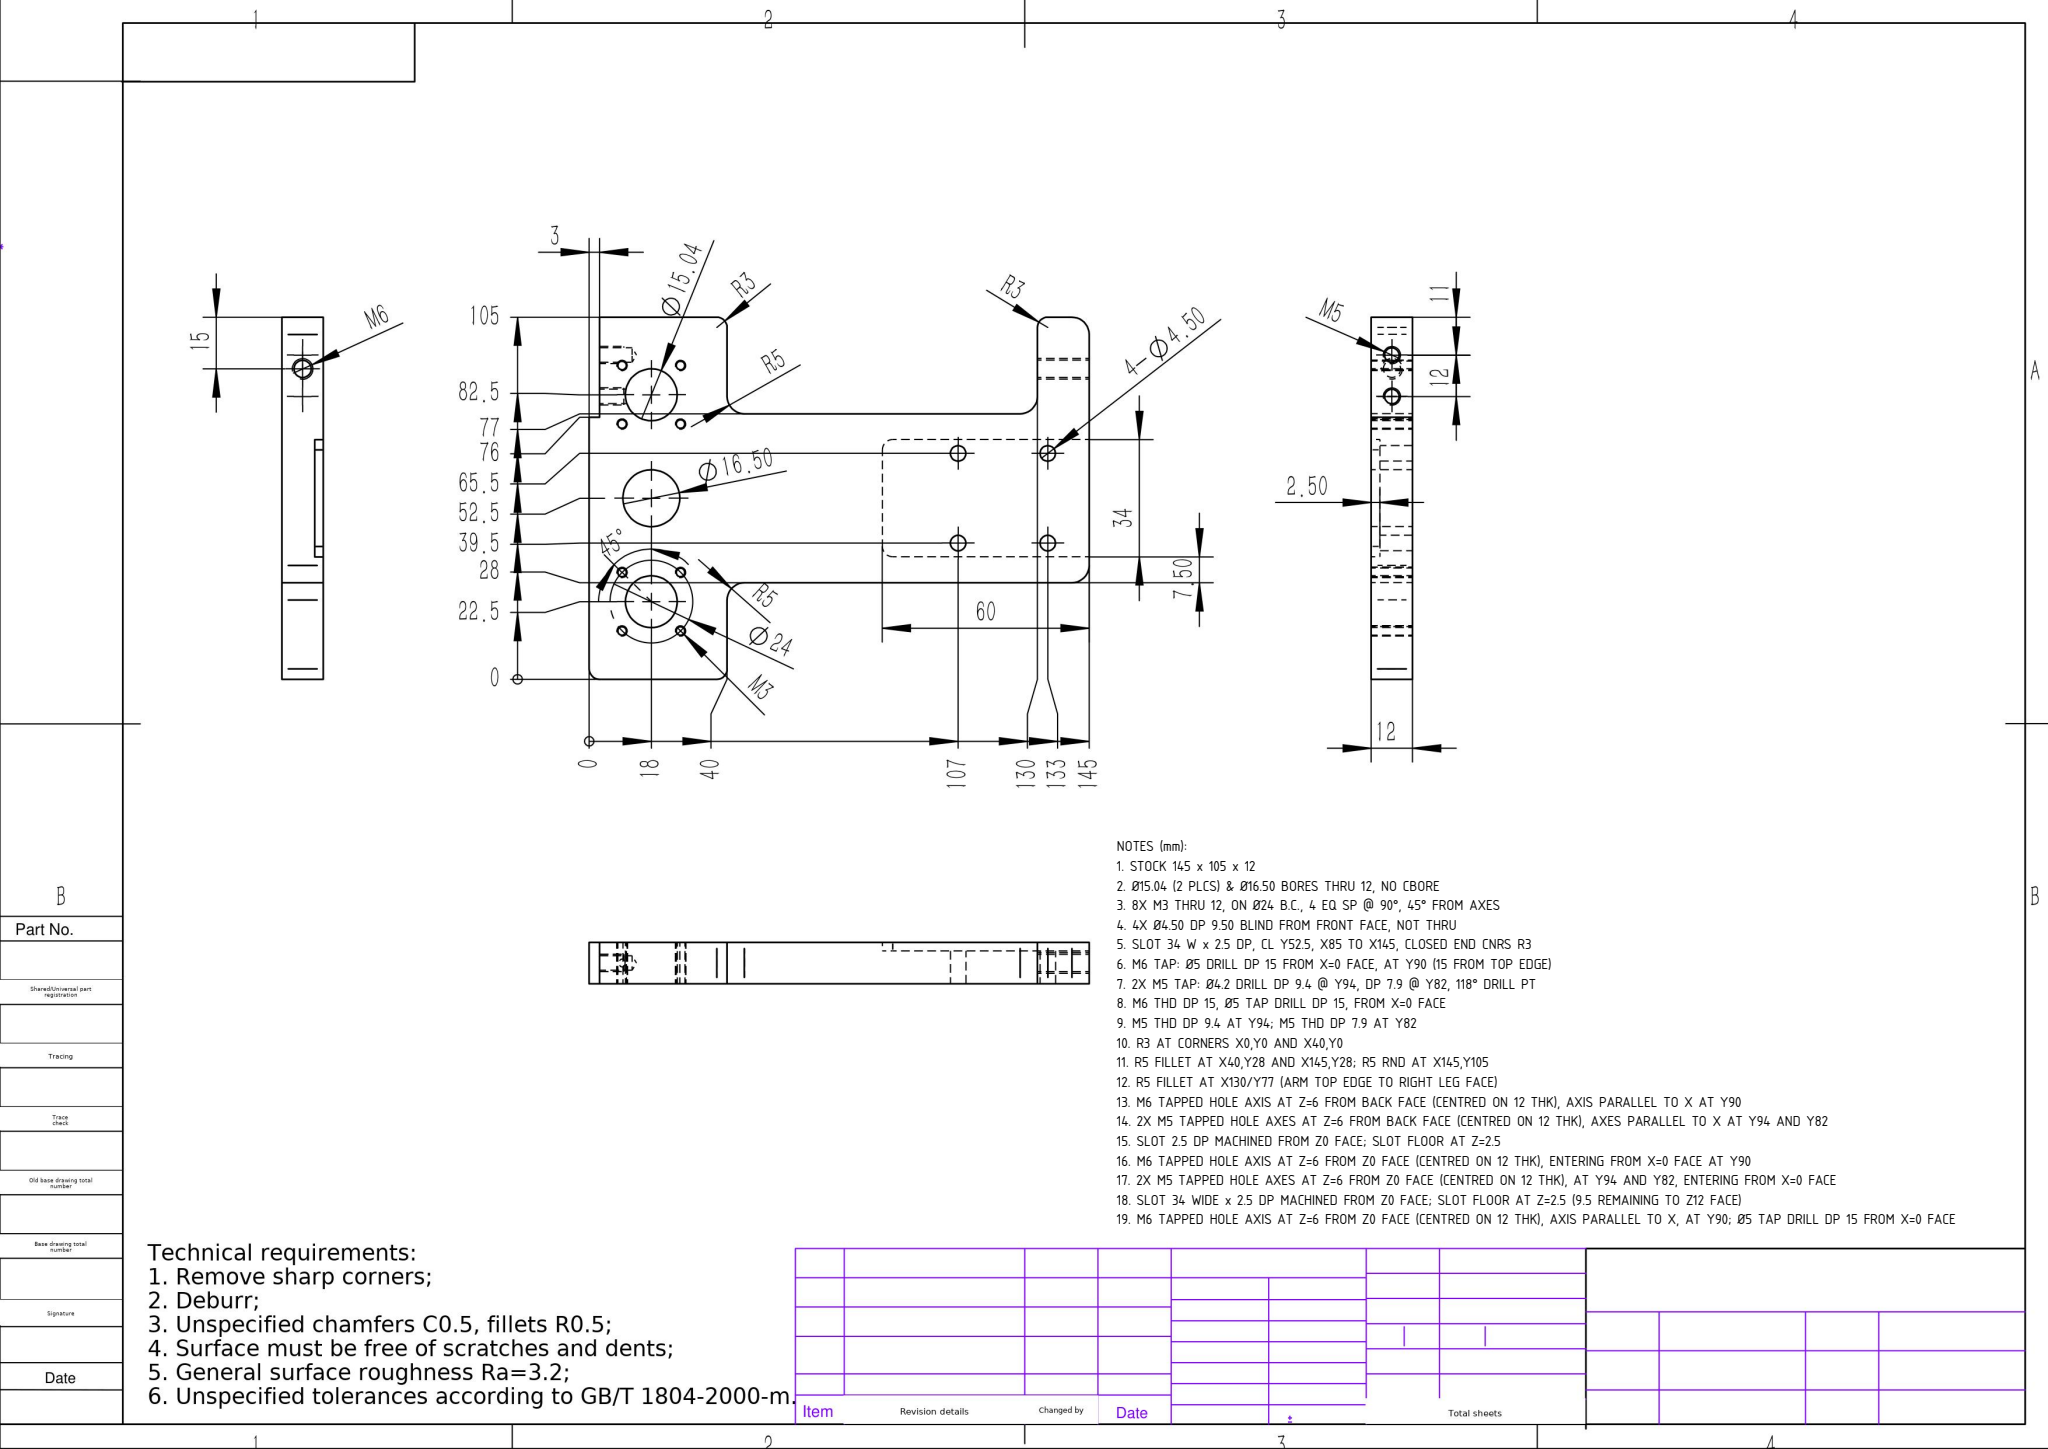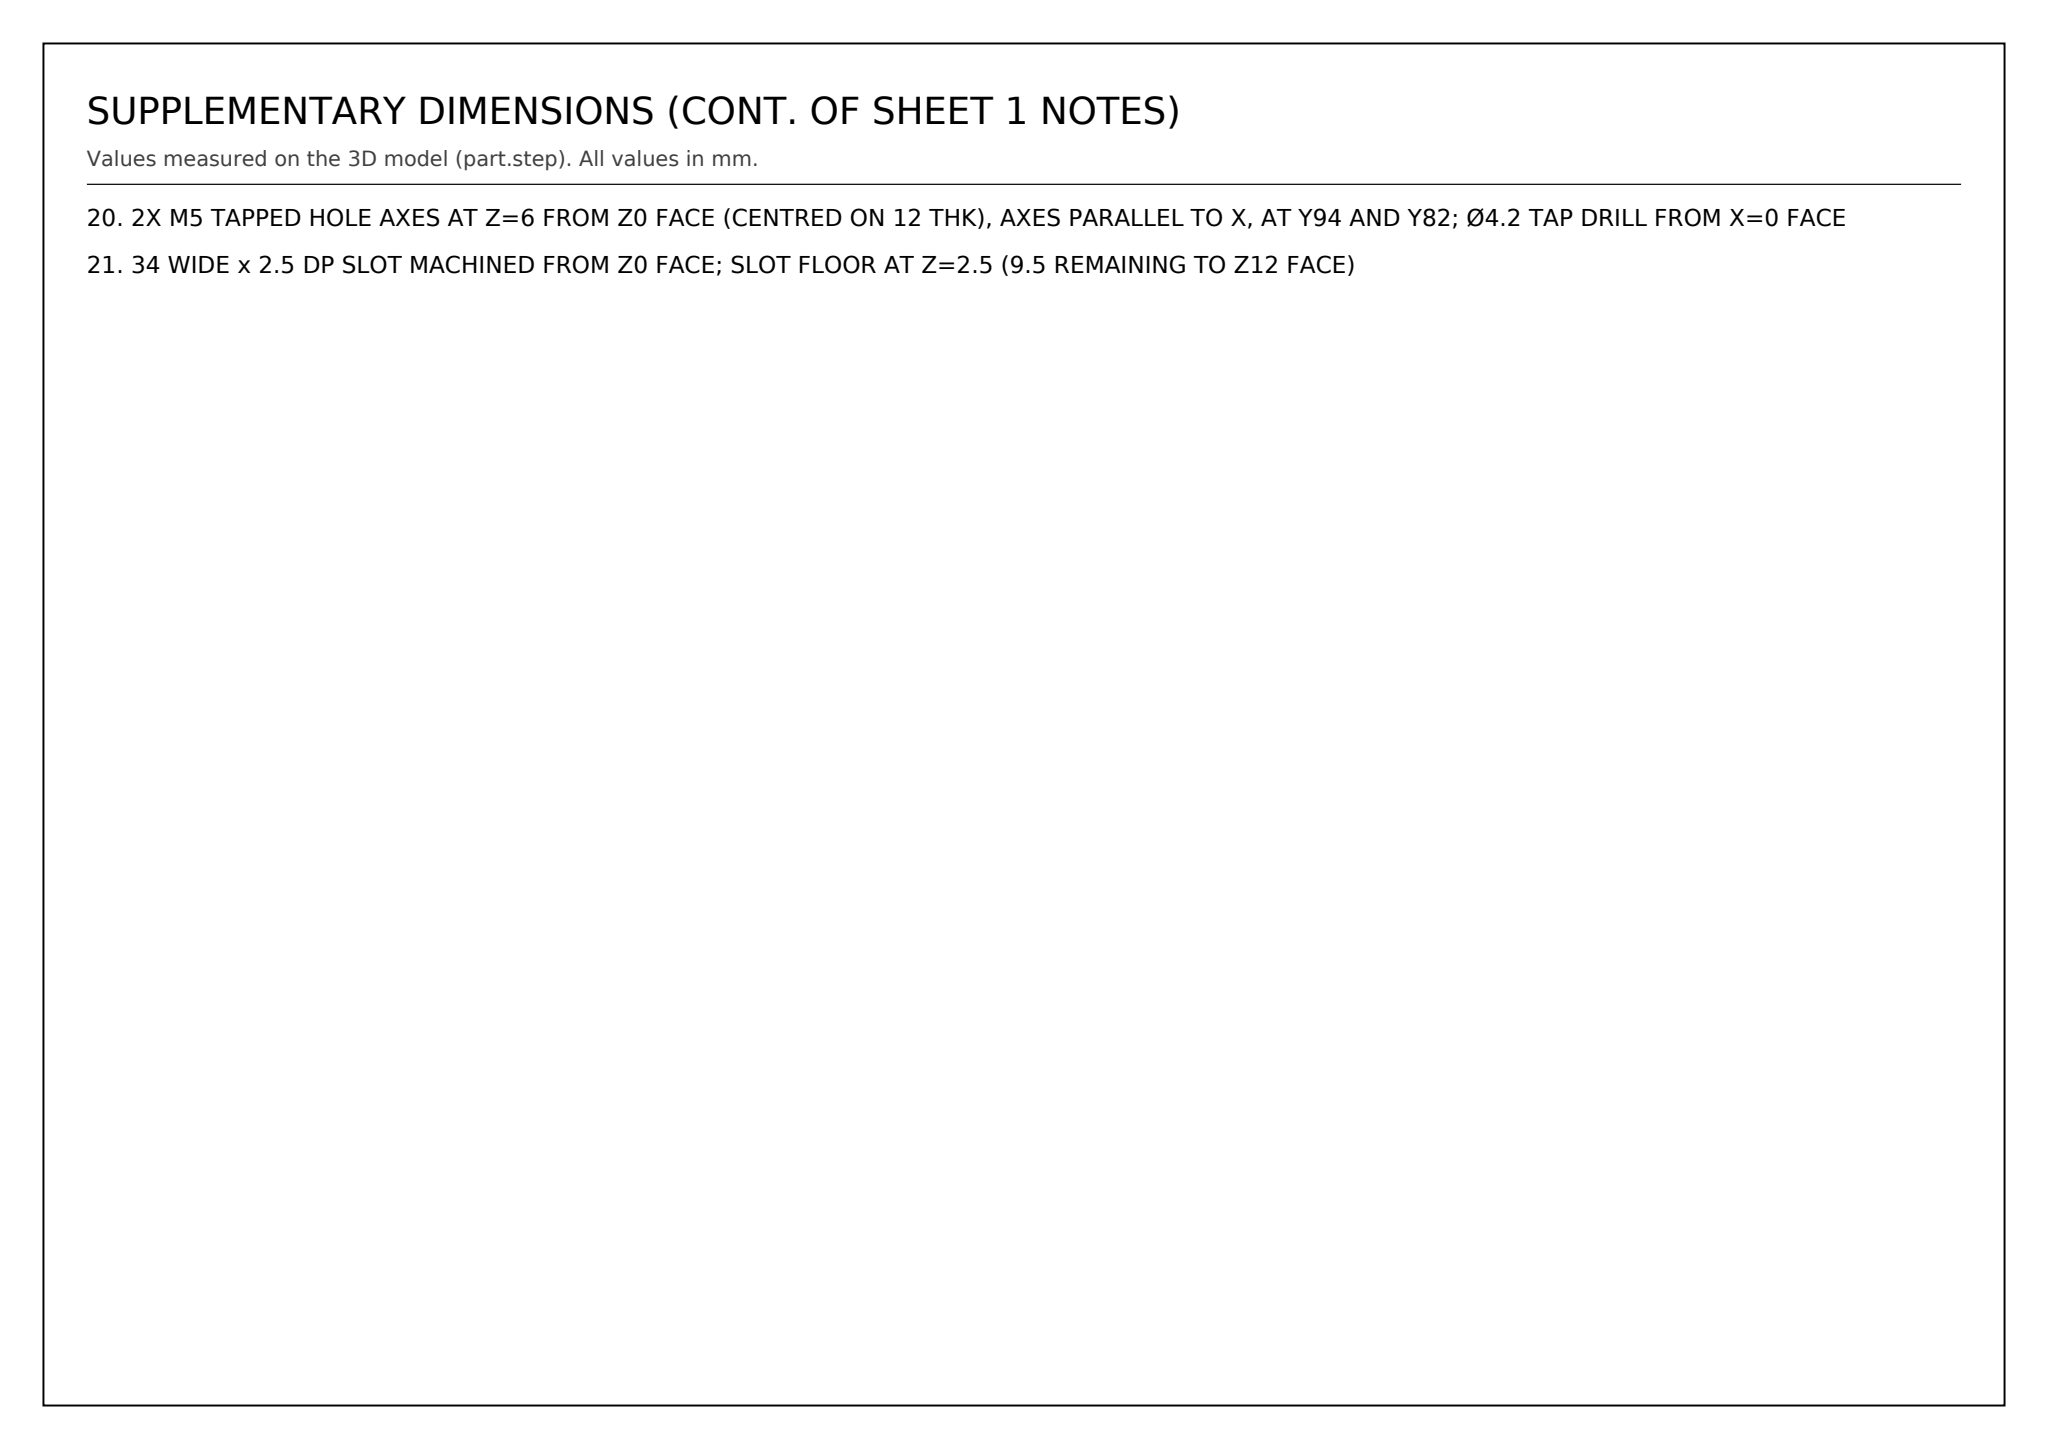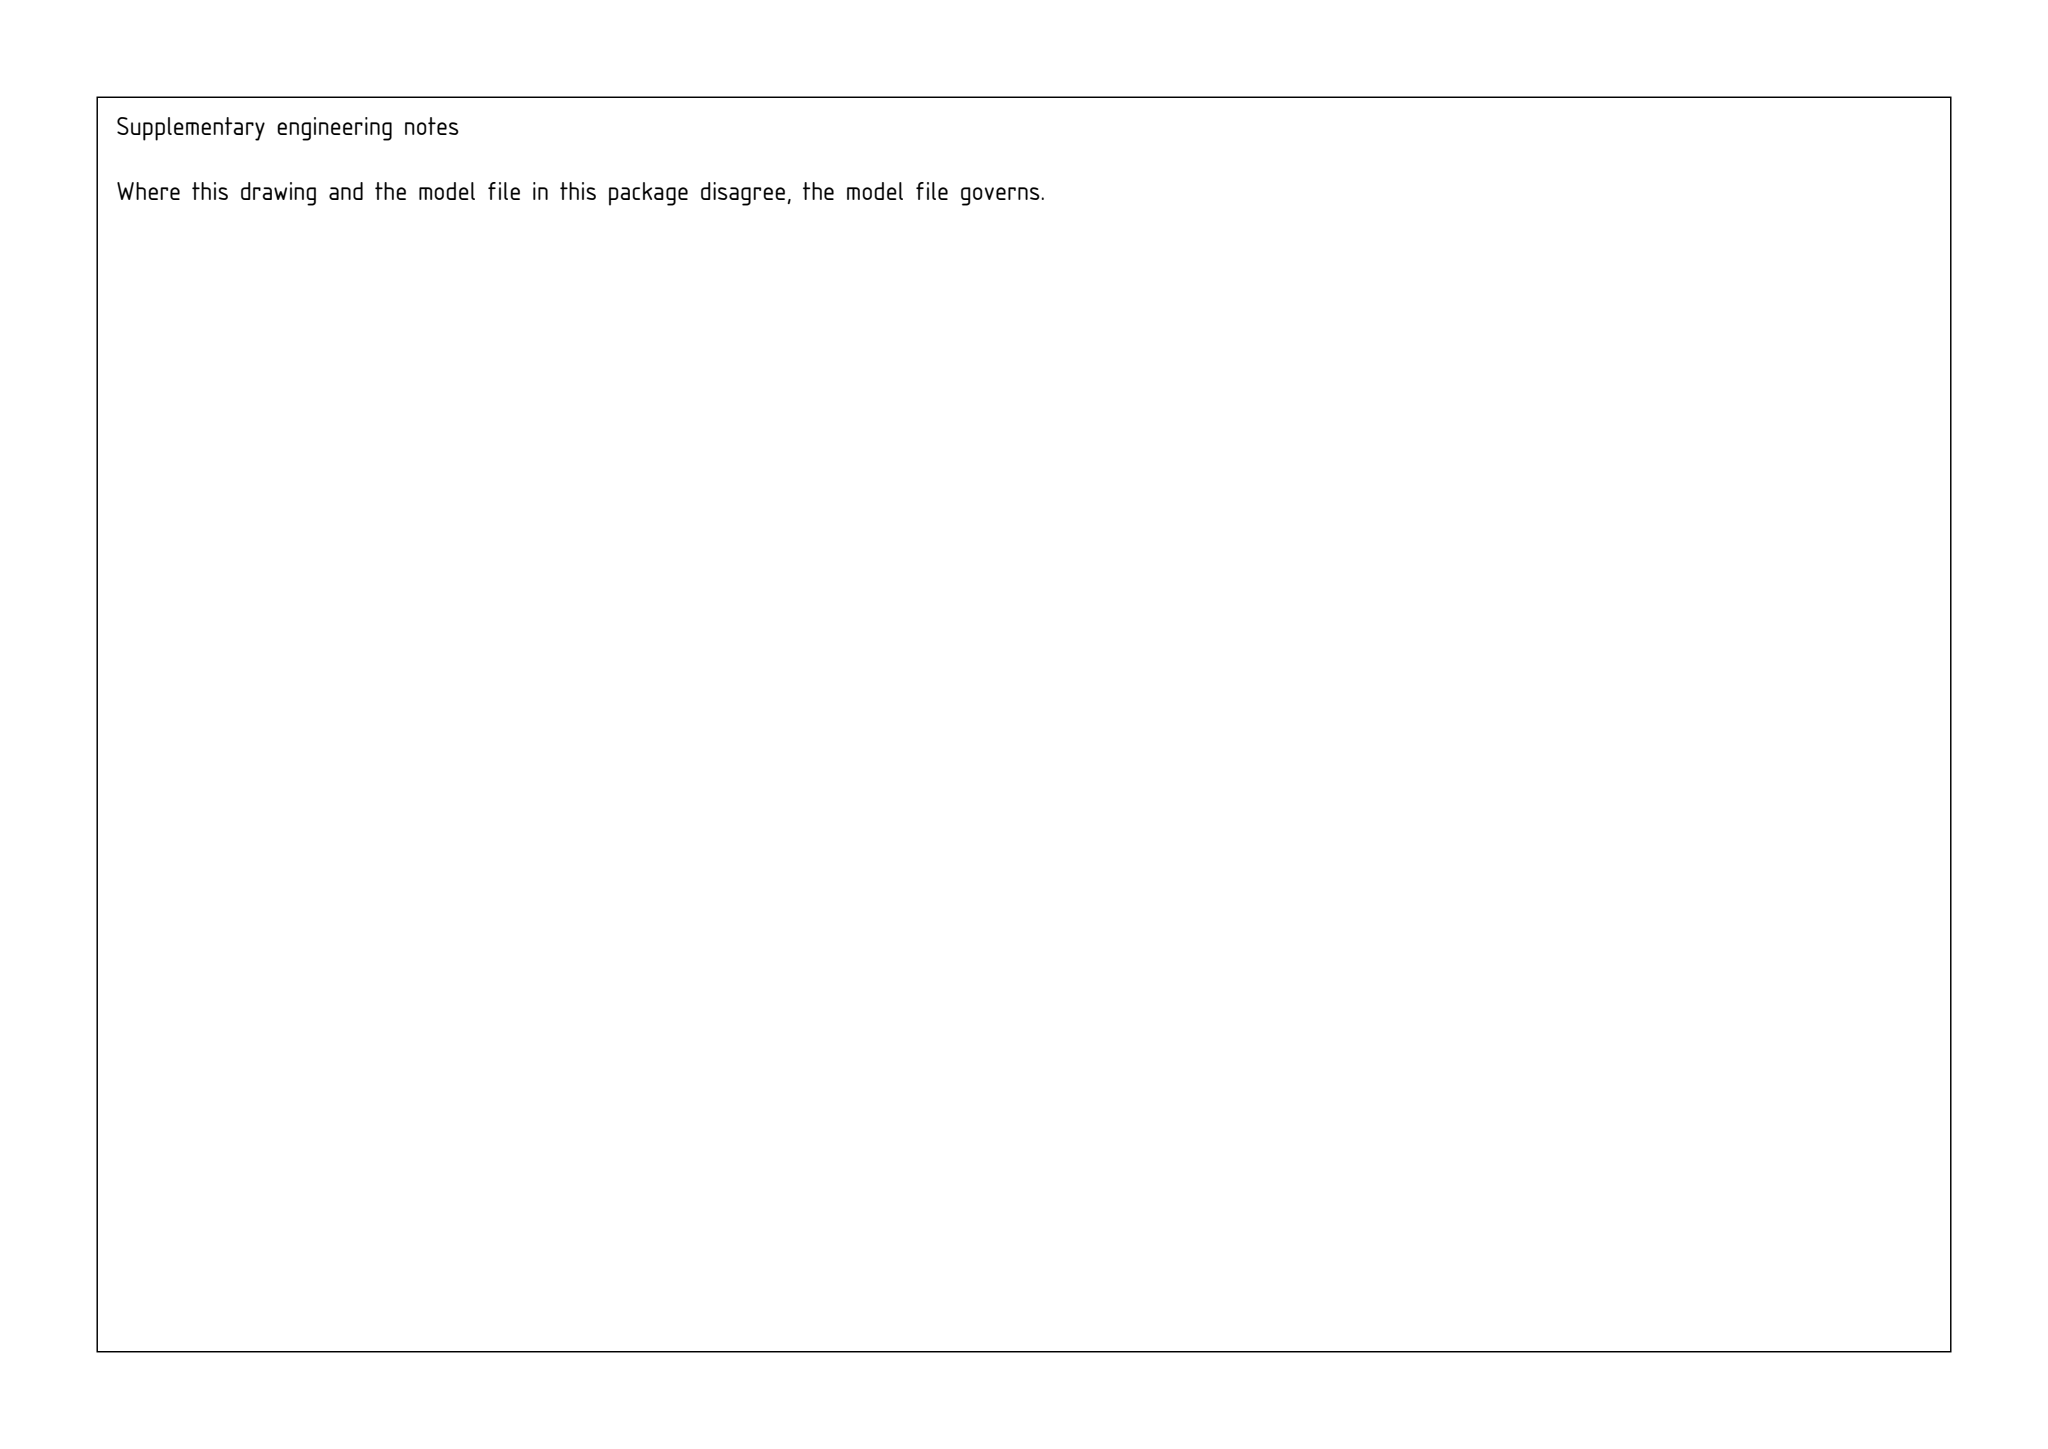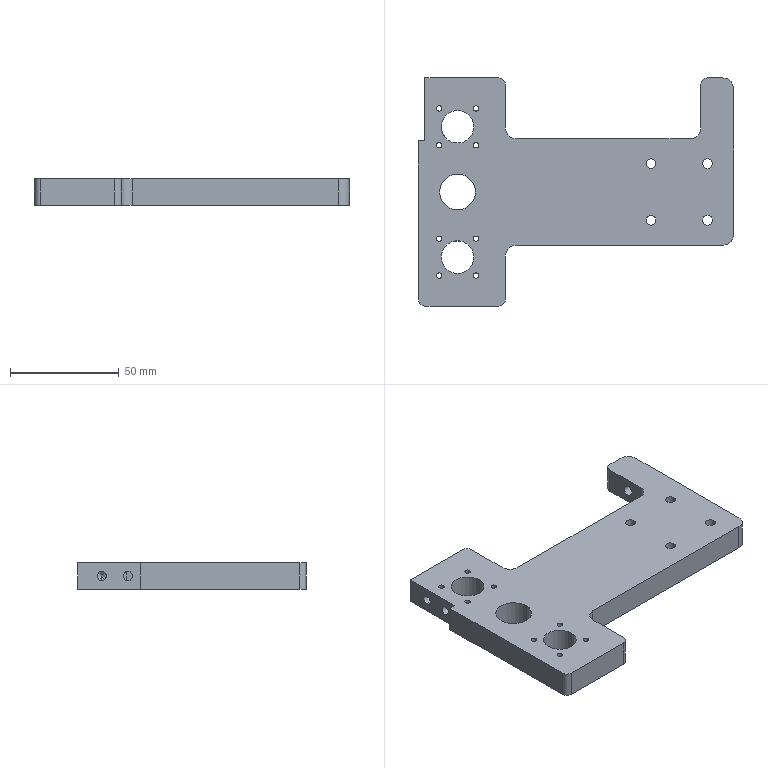Part | SolidWorks | mm | 1 solid | 67 faces | box 145 x 105 x 12 mm | volume 102577 mm3 | cylinder 47 | plane 18 | cone 2 | commonest cylinder face diameters 2.5 x16 4.5 x8 6 x6 10 x5 4.2 x4 15.04 x4 5 x2 16.5 x2
Drawing notes:
STOCK 145 x 105 x 12 | from the solid: bbox_xyz [145.0,105.0,12.0]
Ø15.04 (2 PLCS) & Ø16.50 BORES THRU 12, NO CBORE | from the solid: 15.04 z-cyls L=12 at (18,22.5) & (18,82.5); 16.5 z-cyl L=12 at (18,52.5); no larger coaxial cyl
8X M3 THRU 12, ON Ø24 B.C., 4 EQ SP @ 90°, 45° FROM AXES | from the solid: Ø2.5 z-holes L=12 at (9.51/26.49, 14.01/30.99) and (9.51/26.49, 74.01/90.99): ±8.49,±8.49 = R12 at 45°
4X Ø4.50 DP 9.50 BLIND FROM FRONT FACE, NOT THRU | from the solid: 4.5 z-cyls L=9.5 at (107,39.5),(107,65.5),(133,39.5),(133,65.5); plate thk 12
SLOT 34 W x 2.5 DP, CL Y52.5, X85 TO X145, CLOSED END CNRS R3 | from the solid: planes y=35.5 & 69.5 (34 apart, CL 52.5), z=2.5 floor, x=85 wall; Ø6 z-cyls L=2.5 at (88,38.5),(88,66.5)
M6 TAP: Ø5 DRILL DP 15 FROM X=0 FACE, AT Y90 (15 FROM TOP EDGE) | from the solid: [5.0,x,[null,90.0,6.0],15.0]; bbox Y=105 so Y90 = 15 from top
2X M5 TAP: Ø4.2 DRILL DP 9.4 @ Y94, DP 7.9 @ Y82, 118° DRILL PT | from the solid: [4.2,x,[null,94.0,6.0],9.4,2]; [4.2,x,[null,82.0,6.0],7.94]; cones[118.0,4.2,2]
M6 THD DP 15, Ø5 TAP DRILL DP 15, FROM X=0 FACE | from the solid: Ø5 cyl, axis X, at Y90 Z6, length 15 (only X-axis Ø5 feature)
M5 THD DP 9.4 AT Y94; M5 THD DP 7.9 AT Y82 | from the solid: Ø4.2 cyls axis X at Y94 Z6 L9.4; at Y82 Z6 L7.94/7.65 + 118° pts
R3 AT CORNERS X0,Y0 AND X40,Y0 | from the solid: Ø6 z-cyls at (3,3) and (37,3), L12 = R3 rounds on X0Y0 & X40Y0
R5 FILLET AT X40,Y28 AND X145,Y28; R5 RND AT X145,Y105 | from the solid: Ø10 z-cyls at (45,23),(140,33),(140,100), L12 = R5 at those corners
R5 FILLET AT X130/Y77 (ARM TOP EDGE TO RIGHT LEG FACE) | from the solid: axis_planes x=130 and y=77 intersect; inside corner matches R5 rounds listed elsewhere (X40,Y77 and X40,Y28)
M6 TAPPED HOLE AXIS AT Z=6 FROM BACK FACE (CENTRED ON 12 THK), AXIS PARALLEL TO X AT Y90 | from the solid: cylinder dia 5.0, axis x, pos [y=90, z=6], length 15.0
2X M5 TAPPED HOLE AXES AT Z=6 FROM BACK FACE (CENTRED ON 12 THK), AXES PARALLEL TO X AT Y94 AND Y82 | from the solid: cylinders dia 4.2, axis x, pos [y=94, z=6] len 9.4 and [y=82, z=6] len 7.94/7.65
SLOT 2.5 DP MACHINED FROM Z0 FACE; SLOT FLOOR AT Z=2.5 | from the solid: axis plane z=2.5 and 6.0 dia cylinders at z-length 2.5 (slot end radii at x88, y38.5/66.5)
M6 TAPPED HOLE AXIS AT Z=6 FROM Z0 FACE (CENTRED ON 12 THK), ENTERING FROM X=0 FACE AT Y90 | from the solid: cylinder dia 5.0, axis x, pos_other_axes [null,90.0,6.0], length 15.0
2X M5 TAPPED HOLE AXES AT Z=6 FROM Z0 FACE (CENTRED ON 12 THK), AT Y94 AND Y82, ENTERING FROM X=0 FACE | from the solid: cylinders dia 4.2, axis x, pos_other_axes [null,94.0,6.0] and [null,82.0,6.0]
SLOT 34 WIDE x 2.5 DP MACHINED FROM Z0 FACE; SLOT FLOOR AT Z=2.5 (9.5 REMAINING TO Z12 FACE) | from the solid: axis_planes z=0.0, z=2.5, z=12.0; slot-end cylinders dia 6.0 at [88,38.5] and [88,66.5] length 2.5
M6 TAPPED HOLE AXIS AT Z=6 FROM Z0 FACE (CENTRED ON 12 THK), AXIS PARALLEL TO X, AT Y90; Ø5 TAP DRILL DP 15 FROM X=0 FACE | from the solid: cylinder dia 5.0, axis x, pos [y=90, z=6], length 15
2X M5 TAPPED HOLE AXES AT Z=6 FROM Z0 FACE (CENTRED ON 12 THK), AXES PARALLEL TO X, AT Y94 AND Y82; Ø4.2 TAP DRILL FROM X=0 FACE | from the solid: cylinders dia 4.2, axis x, pos [y=94, z=6] and [y=82, z=6]
34 WIDE x 2.5 DP SLOT MACHINED FROM Z0 FACE; SLOT FLOOR AT Z=2.5 (9.5 REMAINING TO Z12 FACE) | from the solid: axis_plane z=0 and z=2.5; slot end cylinders dia 6.0 axis z at [88,38.5] and [88,66.5] length 2.5
build123d program:
from build123d import *

# Parameters (mm, degrees)
SKETCH1_W             = 145
SKETCH1_H             = 105
BOSS_EXTRUDE1_DEPTH   = 12
SKETCH3_W             = 5
SKETCH3_H             = 34
CUT_EXTRUDE2_DEPTH    = 60
SKETCH4_R             = 2.25
CUT_EXTRUDE3_DEPTH    = 91.313
SKETCH7_R             = 8.25
CUT_EXTRUDE4_DEPTH    = 91.313
SKETCH8_R             = 7.52
CUT_EXTRUDE5_DEPTH    = 91.313
SKETCH9_W             = 210
SKETCH9_H             = 56
CUT_EXTRUDE6_DEPTH    = 91.313
FILLET1_R             = 5
FILLET2_R             = 3
M5_TAPPED_HOLE2_D     = 4.2
M5_TAPPED_HOLE2_DEPTH = 12.4
M5_TAPPED_HOLE2_TIP   = 1.262
SKETCH12_W            = 3
SKETCH12_H            = 29
CUT_EXTRUDE7_DEPTH    = 91.313
SKETCH13_W            = 15
SKETCH13_H            = 12
BOSS_EXTRUDE2_DEPTH   = 28
FILLET3_R             = 5
FILLET4_R             = 5
FILLET5_R             = 3
M6_TAPPED_HOLE1_D     = 5
M6_TAPPED_HOLE1_DEPTH = 25
M6_TAPPED_HOLE1_TIP   = 1.502
M3_TAPPED_HOLE1_D     = 2.5
FILLET6_R             = 3


with BuildPart() as part:
    # Sketch1 → Boss-Extrude1 (new body)
    with BuildSketch(Plane.XY):
        Rectangle(SKETCH1_W, SKETCH1_H)
    extrude(amount=BOSS_EXTRUDE1_DEPTH)

    # Sketch3 → Cut-Extrude2 (cut)
    with BuildSketch(Plane(origin=(72.5, 0, 0), x_dir=(0, 0, -1), z_dir=(1, 0, 0))):
        Rectangle(SKETCH3_W, SKETCH3_H)
    extrude(amount=-CUT_EXTRUDE2_DEPTH, mode=Mode.SUBTRACT)

    # Sketch4 → Cut-Extrude3 (cut, through all)
    with BuildSketch(Plane.XY.offset(12)):
        with Locations((34.5, 13)):
            Circle(SKETCH4_R)
        with Locations((60.5, 13)):
            Circle(SKETCH4_R)
        with Locations((34.5, -13)):
            Circle(SKETCH4_R)
        with Locations((60.5, -13)):
            Circle(SKETCH4_R)
    extrude(amount=-CUT_EXTRUDE3_DEPTH, mode=Mode.SUBTRACT)

    # Sketch7 → Cut-Extrude4 (cut, through all)
    with BuildSketch(Plane.XY.offset(12)):
        with Locations((-54.5, 0)):
            Circle(SKETCH7_R)
    extrude(amount=-CUT_EXTRUDE4_DEPTH, mode=Mode.SUBTRACT)

    # Sketch8 → Cut-Extrude5 (cut, through all)
    with BuildSketch(Plane.XY.offset(12)):
        with Locations((-54.5, 30)):
            Circle(SKETCH8_R)
        with Locations(Location((-54.5, -30, 0), (0, 0, 180))):
            Circle(SKETCH8_R)
    extrude(amount=-CUT_EXTRUDE5_DEPTH, mode=Mode.SUBTRACT)

    # Sketch9 → Cut-Extrude6 (cut, through all)
    with BuildSketch(Plane.XY.offset(12)):
        with Locations((72.5, 52.5)):
            Rectangle(SKETCH9_W, SKETCH9_H)
        with Locations((72.5, -52.5)):
            Rectangle(SKETCH9_W, SKETCH9_H)
    extrude(amount=-CUT_EXTRUDE6_DEPTH, mode=Mode.SUBTRACT)

    # Fillet1
    fillet1_edges = [part.edges().sort_by_distance(p)[0] for p in [
        (-32.5, 24.5, 6),
        (-32.5, -24.5, 6),
    ]]
    fillet(fillet1_edges, radius=FILLET1_R)

    # Fillet2
    fillet2_edges = [part.edges().sort_by_distance(p)[0] for p in [
        (-32.5, 52.5, 6),
        (-72.5, -52.5, 6),
        (-72.5, 52.5, 6),
        (-32.5, -52.5, 6),
    ]]
    fillet(fillet2_edges, radius=FILLET2_R)

    # M5 Tapped Hole2
    with Locations(Plane.ZY.offset(72.5)):
        with Locations((6, 29.5), (6, 41.5)):
            Hole(M5_TAPPED_HOLE2_D / 2, depth=M5_TAPPED_HOLE2_DEPTH)
            with Locations((0, 0, -(M5_TAPPED_HOLE2_DEPTH + M5_TAPPED_HOLE2_TIP / 2))):  # 118° drill point
                Cone(0, M5_TAPPED_HOLE2_D / 2, M5_TAPPED_HOLE2_TIP, mode=Mode.SUBTRACT)

    # Sketch12 → Cut-Extrude7 (cut, through all)
    with BuildSketch(Plane.XY.offset(12)):
        with Locations((-71, 38)):
            Rectangle(SKETCH12_W, SKETCH12_H)
    extrude(amount=-CUT_EXTRUDE7_DEPTH, mode=Mode.SUBTRACT)

    # Sketch13 → Boss-Extrude2 (add)
    with BuildSketch(Plane(origin=(0, 24.5, 0), x_dir=(1, 0, 0), z_dir=(0, 1, 0))):
        with Locations((65, -6)):
            Rectangle(SKETCH13_W, SKETCH13_H)
    extrude(amount=BOSS_EXTRUDE2_DEPTH)

    # Fillet3
    fillet3_edges = [part.edges().sort_by_distance(p)[0] for p in [
        (57.5, 24.5, 6),
    ]]
    fillet(fillet3_edges, radius=FILLET3_R)

    # Fillet4
    fillet4_edges = [part.edges().sort_by_distance(p)[0] for p in [
        (72.5, 52.5, 6),
        (72.5, -24.5, 6),
    ]]
    fillet(fillet4_edges, radius=FILLET4_R)

    # Fillet5
    fillet5_edges = [part.edges().sort_by_distance(p)[0] for p in [
        (57.5, 52.5, 6),
    ]]
    fillet(fillet5_edges, radius=FILLET5_R)

    # M6 Tapped Hole1
    with Locations(Plane(origin=(72.5, 0, 0), x_dir=(0, 0, -1), z_dir=(1, 0, 0))):
        with Locations((-6, 37.5)):
            Hole(M6_TAPPED_HOLE1_D / 2, depth=M6_TAPPED_HOLE1_DEPTH)
            with Locations((0, 0, -(M6_TAPPED_HOLE1_DEPTH + M6_TAPPED_HOLE1_TIP / 2))):  # 118° drill point
                Cone(0, M6_TAPPED_HOLE1_D / 2, M6_TAPPED_HOLE1_TIP, mode=Mode.SUBTRACT)

    # M3 Tapped Hole1 (through all)
    with Locations(Plane(origin=(0, 0, 0), x_dir=(-1, 0, 0), z_dir=(0, 0, -1))):
        with Locations((46.015, 21.515), (46.015, 38.485), (62.985, 38.485), (62.985, 21.515), (46.015, -21.515), (62.985, -21.515), (46.015, -38.485), (62.985, -38.485)):
            Hole(M3_TAPPED_HOLE1_D / 2)

    # Fillet6
    fillet6_edges = [part.edges().sort_by_distance(p)[0] for p in [
        (12.5, -17, 1.25),
        (12.5, 17, 1.25),
    ]]
    fillet(fillet6_edges, radius=FILLET6_R)


solid = part.part